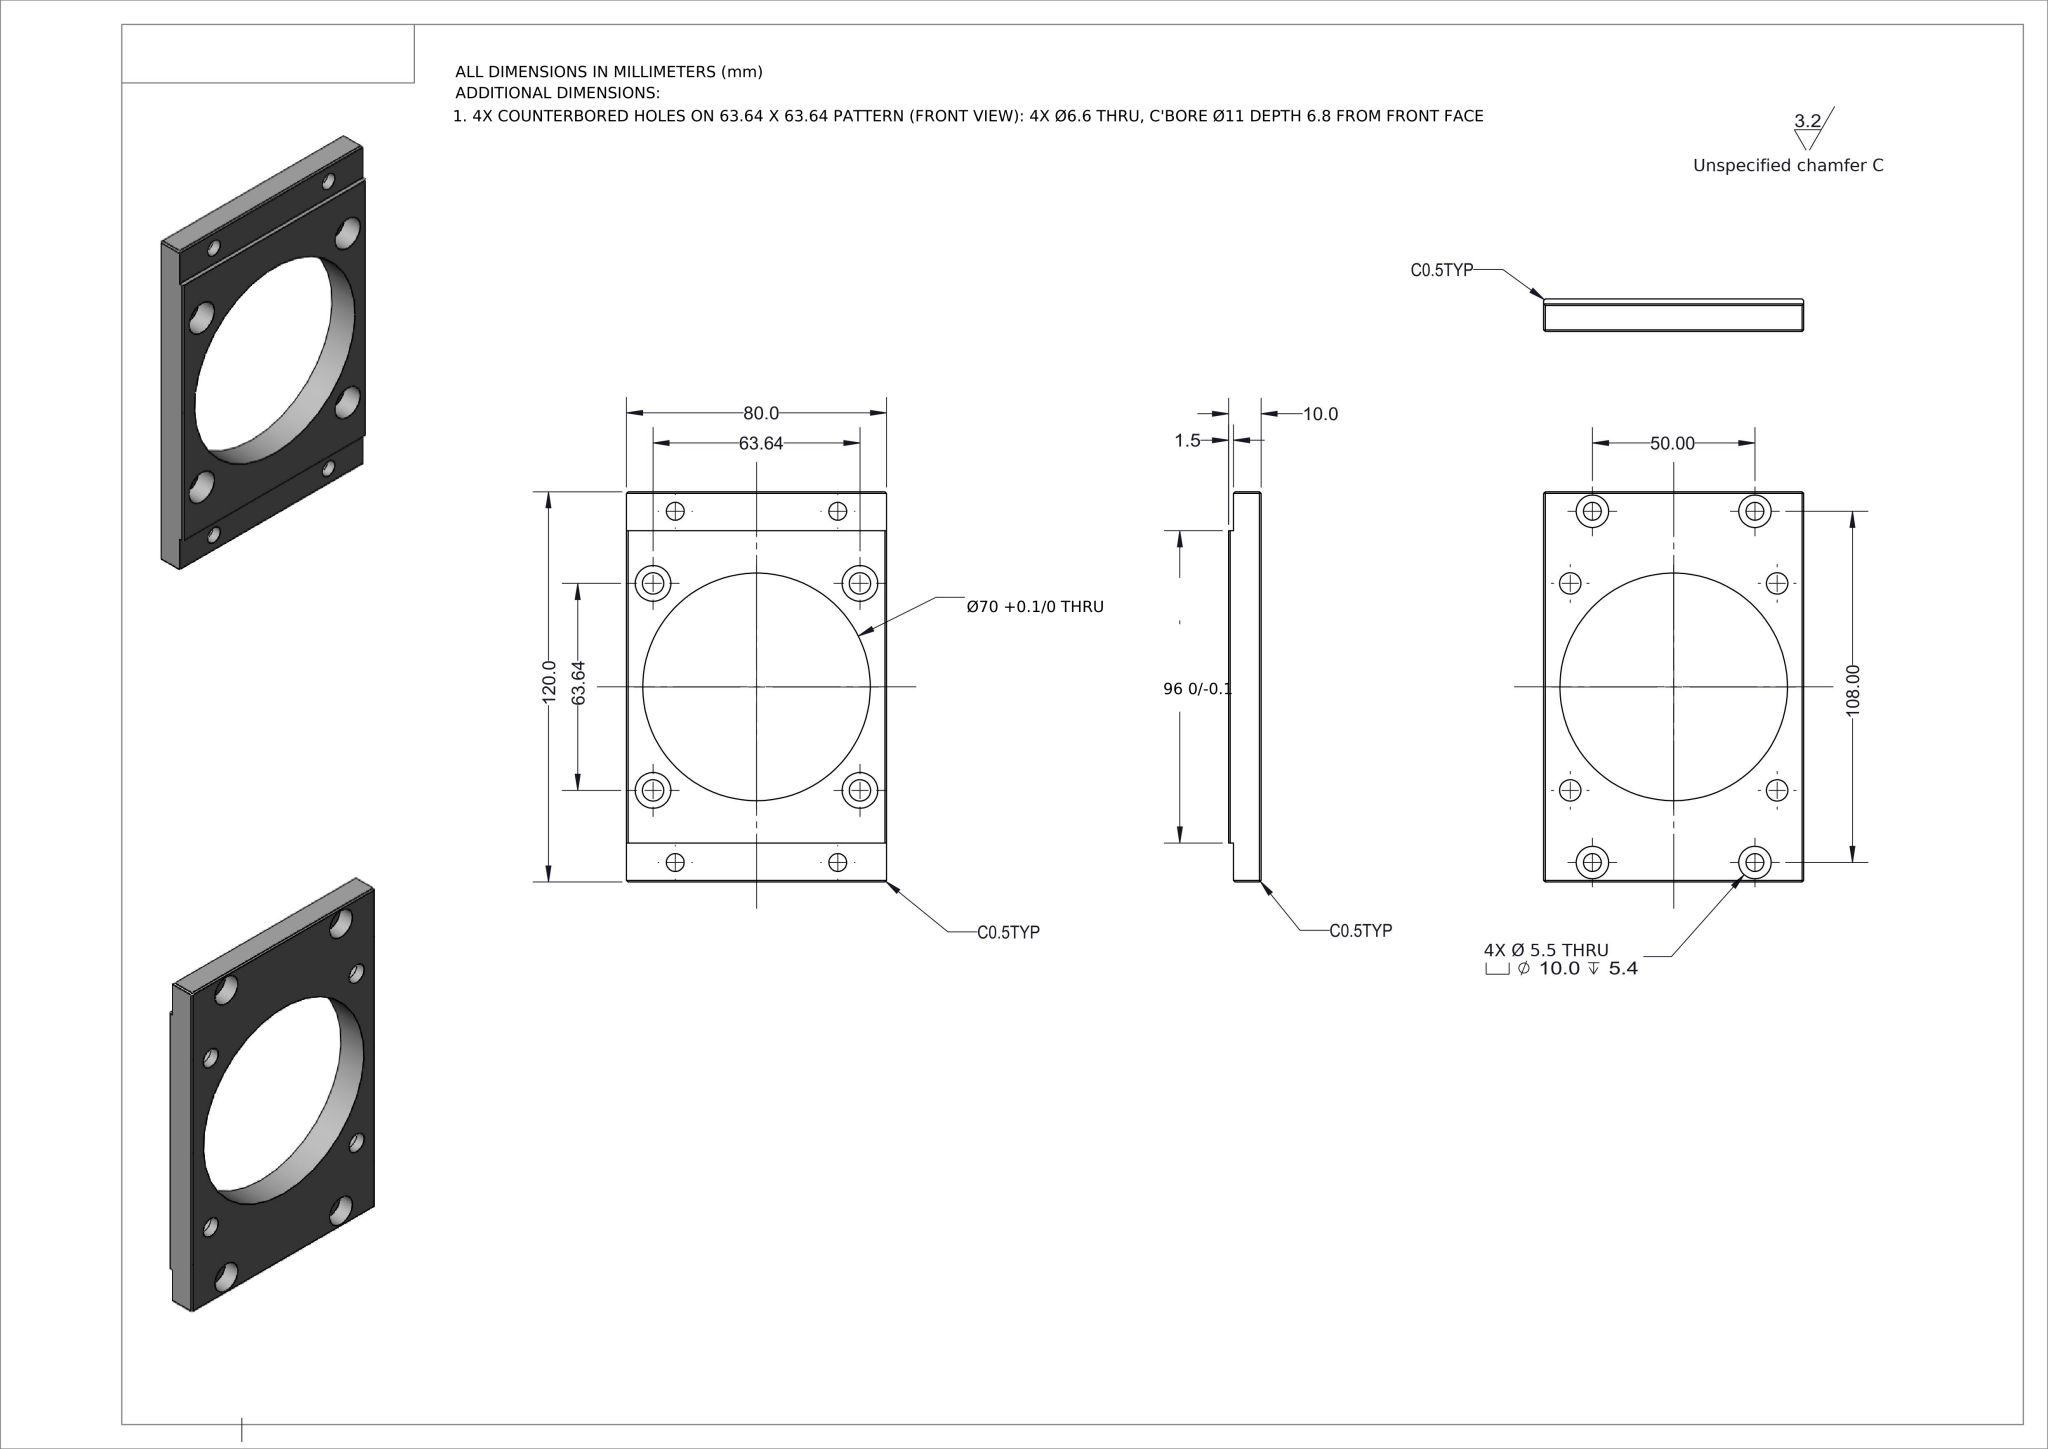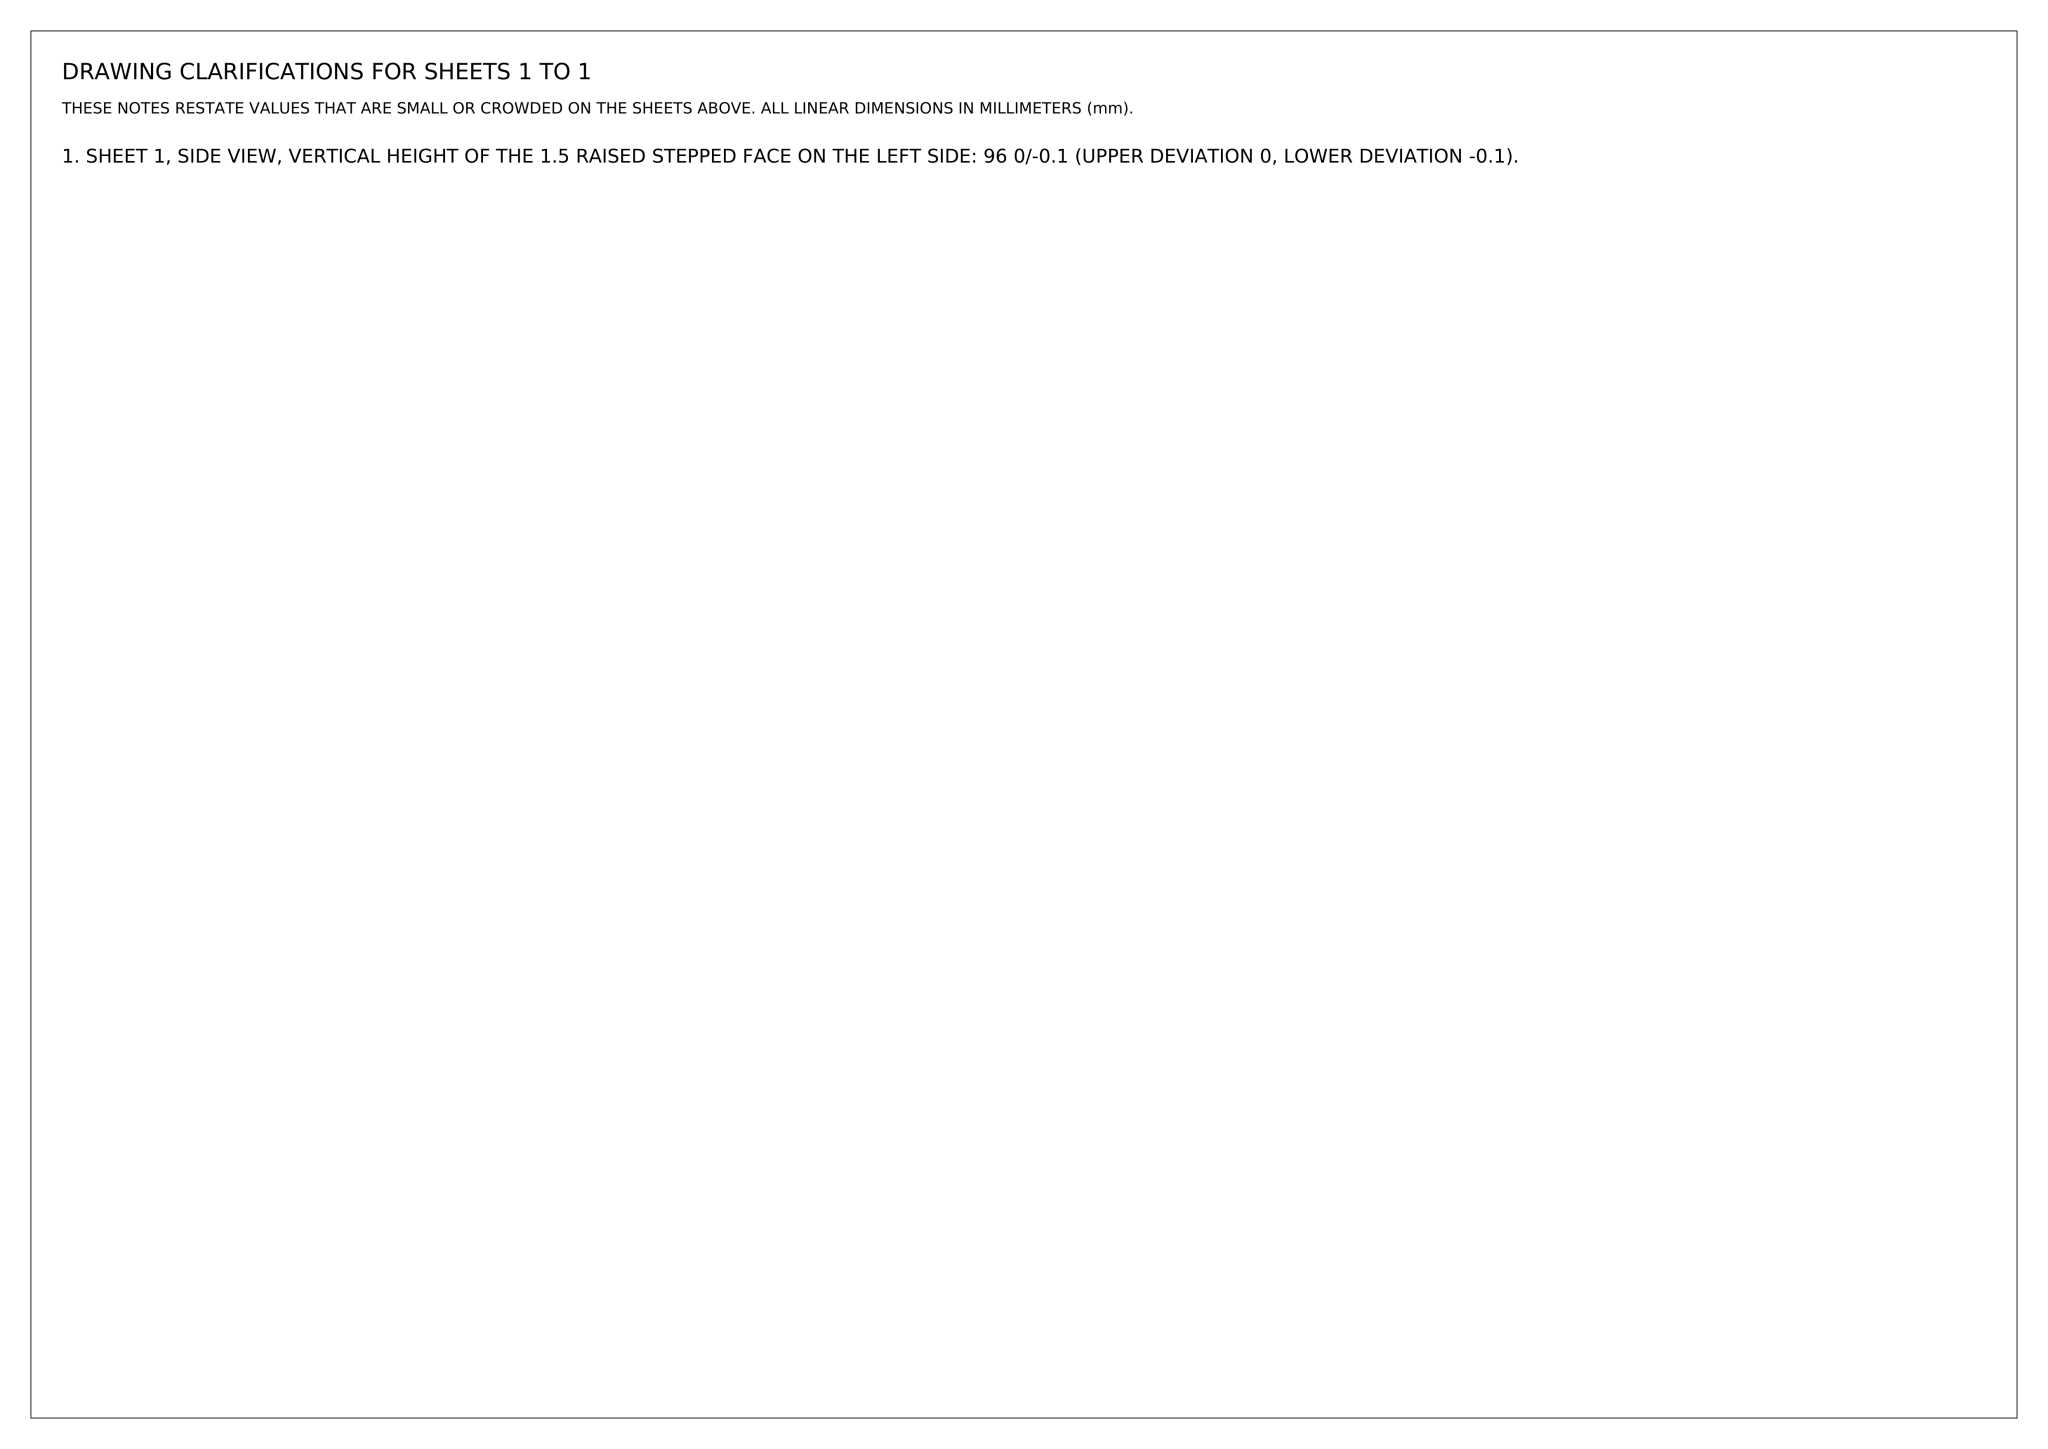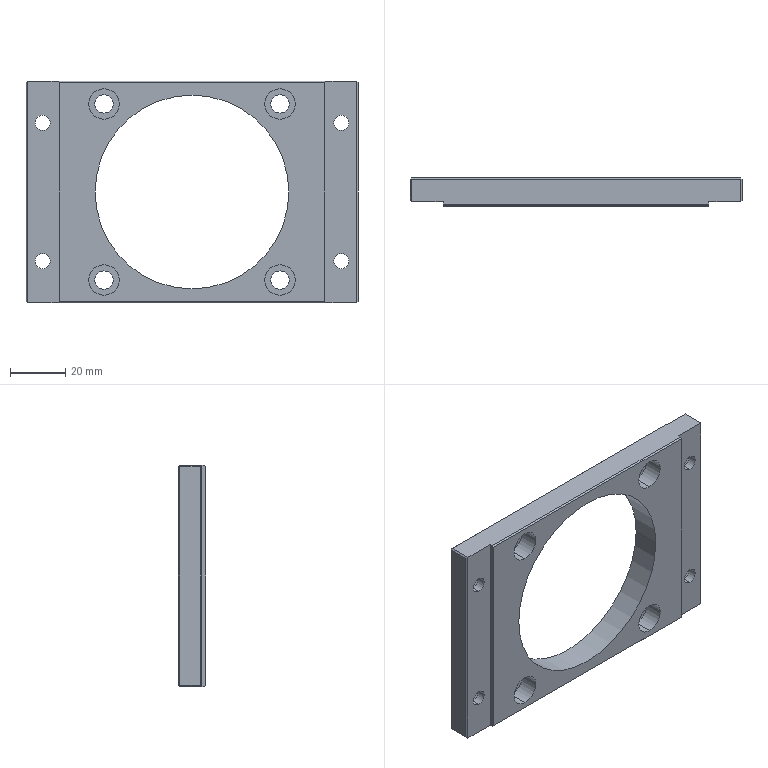Part | NX | mm | 1 solid | 68 faces | box 120 x 10 x 80 mm | volume 49524 mm3 | cylinder 34 | plane 34 | commonest cylinder face diameters 11 x8 6.6 x8 10 x8 5.5 x8 70 x2